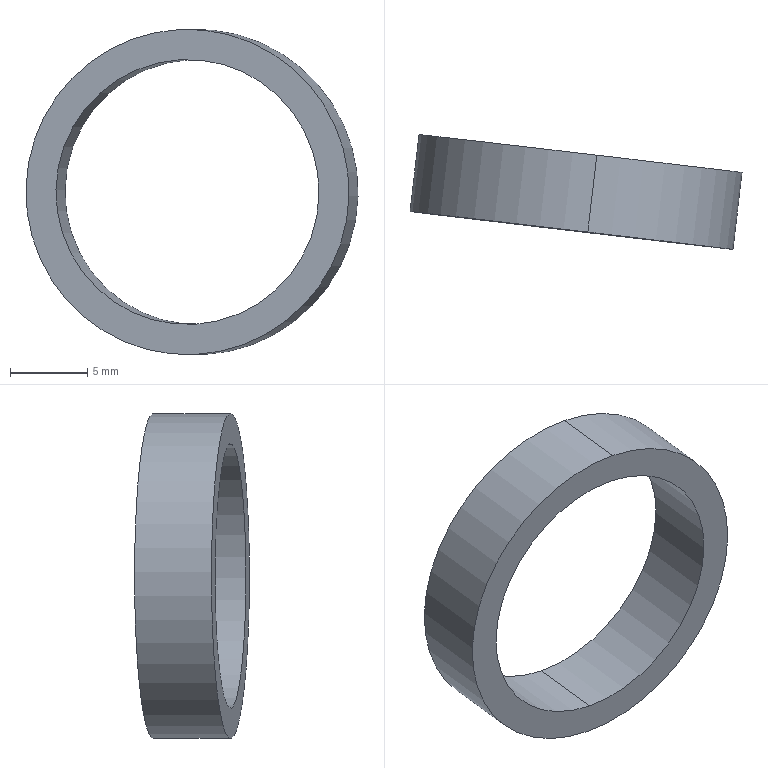Component | SolidWorks | 8TC-A17001-91-00UpperAndLowerPressAssembly-1_8TC-A17001-91-01Spacer-1 | 1 solid | 6 faces | box 21.44 x 7.42 x 21 mm | volume 584 mm3 | cylinder 4 | plane 2 | commonest cylinder face diameters 17.1 x2 21 x2 | material A3
build123d program:
from build123d import *

# Parameters (mm, degrees)
SKETCH1_R           = 10.5
SKETCH1_R_2         = 8.55
BOSS_EXTRUDE1_DEPTH = 5


with BuildPart() as part:
    # Sketch1 → Boss-Extrude1 (new body)
    with BuildSketch(Plane(origin=(0, 0, 0), x_dir=(1, 0, 0), z_dir=(0, 1, 0))):
        with Locations(Location((0, 0, 0), (0, 0, 270))):
            Circle(SKETCH1_R)
        with Locations(Location((0, 0, 0), (0, 0, 270))):
            Circle(SKETCH1_R_2, mode=Mode.SUBTRACT)
    extrude(amount=BOSS_EXTRUDE1_DEPTH)


solid = part.part

# Placed as in the assembly
solid = solid.moved(Location((1.253, -81.585, -52), (-35.549, -78.578, 143.907)))
STEP:
#1=CARTESIAN_POINT('',(0.0156,-3.208,-2.382));
#2=VERTEX_POINT('',#1);
#3=CARTESIAN_POINT('',(0.08309,-3.216,-1.712));
#4=VERTEX_POINT('',#3);
#5=CARTESIAN_POINT('',(0.04935,-3.212,-2.047));
#6=DIRECTION('',(0.1167,0.9932,-0.));
#7=DIRECTION('',(0.1002,-0.01178,0.9949));
#8=AXIS2_PLACEMENT_3D('',#5,#6,#7);
#9=CIRCLE('',#8,0.3366);
#10=EDGE_CURVE('',#2,#4,#9,.T.);
#11=ORIENTED_EDGE('',*,*,#10,.T.);
#12=CARTESIAN_POINT('',(0.06013,-3.411,-1.712));
#13=VERTEX_POINT('',#12);
#14=CARTESIAN_POINT('',(0.08309,-3.216,-1.712));
#15=DIRECTION('',(-0.1167,-0.9932,0.));
#16=VECTOR('',#15,39.37);
#17=LINE('',#14,#16);
#18=EDGE_CURVE('',#4,#13,#17,.T.);
#19=ORIENTED_EDGE('',*,*,#18,.T.);
#20=CARTESIAN_POINT('',(-0.007362,-3.404,-2.382));
#21=VERTEX_POINT('',#20);
#22=CARTESIAN_POINT('',(0.02638,-3.408,-2.047));
#23=DIRECTION('',(0.1167,0.9932,-0.));
#24=DIRECTION('',(0.1002,-0.01178,0.9949));
#25=AXIS2_PLACEMENT_3D('',#22,#23,#24);
#26=CIRCLE('',#25,0.3366);
#27=EDGE_CURVE('',#21,#13,#26,.T.);
#28=ORIENTED_EDGE('',*,*,#27,.F.);
#29=CARTESIAN_POINT('',(0.0156,-3.208,-2.382));
#30=DIRECTION('',(-0.1167,-0.9932,0.));
#31=VECTOR('',#30,39.37);
#32=LINE('',#29,#31);
#33=EDGE_CURVE('',#2,#21,#32,.T.);
#34=ORIENTED_EDGE('',*,*,#33,.F.);
#35=EDGE_LOOP('',(#11,#19,#28,#34));
#36=FACE_OUTER_BOUND('',#35,.T.);
#37=CARTESIAN_POINT('',(0.04935,-3.212,-2.047));
#38=DIRECTION('',(-0.1167,-0.9932,0.));
#39=DIRECTION('',(-0.1002,0.01178,-0.9949));
#40=AXIS2_PLACEMENT_3D('',#37,#38,#39);
#41=CYLINDRICAL_SURFACE('',#40,0.3366);
#42=ADVANCED_FACE('',(#36),#41,.F.);
#43=CARTESIAN_POINT('',(0.09079,-3.217,-1.636));
#44=VERTEX_POINT('',#43);
#45=CARTESIAN_POINT('',(0.007907,-3.207,-2.459));
#46=VERTEX_POINT('',#45);
#47=CARTESIAN_POINT('',(0.04935,-3.212,-2.047));
#48=DIRECTION('',(0.1167,0.9932,-0.));
#49=DIRECTION('',(0.1002,-0.01178,0.9949));
#50=AXIS2_PLACEMENT_3D('',#47,#48,#49);
#51=CIRCLE('',#50,0.4134);
#52=EDGE_CURVE('',#44,#46,#51,.T.);
#53=ORIENTED_EDGE('',*,*,#52,.F.);
#54=CARTESIAN_POINT('',(0.06782,-3.412,-1.636));
#55=VERTEX_POINT('',#54);
#56=CARTESIAN_POINT('',(0.09079,-3.217,-1.636));
#57=DIRECTION('',(-0.1167,-0.9932,0.));
#58=VECTOR('',#57,39.37);
#59=LINE('',#56,#58);
#60=EDGE_CURVE('',#44,#55,#59,.T.);
#61=ORIENTED_EDGE('',*,*,#60,.T.);
#62=CARTESIAN_POINT('',(-0.01506,-3.403,-2.459));
#63=VERTEX_POINT('',#62);
#64=CARTESIAN_POINT('',(0.02638,-3.408,-2.047));
#65=DIRECTION('',(0.1167,0.9932,-0.));
#66=DIRECTION('',(0.1002,-0.01178,0.9949));
#67=AXIS2_PLACEMENT_3D('',#64,#65,#66);
#68=CIRCLE('',#67,0.4134);
#69=EDGE_CURVE('',#55,#63,#68,.T.);
#70=ORIENTED_EDGE('',*,*,#69,.T.);
#71=CARTESIAN_POINT('',(0.007907,-3.207,-2.459));
#72=DIRECTION('',(-0.1167,-0.9932,0.));
#73=VECTOR('',#72,39.37);
#74=LINE('',#71,#73);
#75=EDGE_CURVE('',#46,#63,#74,.T.);
#76=ORIENTED_EDGE('',*,*,#75,.F.);
#77=EDGE_LOOP('',(#53,#61,#70,#76));
#78=FACE_OUTER_BOUND('',#77,.T.);
#79=CARTESIAN_POINT('',(0.04935,-3.212,-2.047));
#80=DIRECTION('',(-0.1167,-0.9932,0.));
#81=DIRECTION('',(-0.1002,0.01178,-0.9949));
#82=AXIS2_PLACEMENT_3D('',#79,#80,#81);
#83=CYLINDRICAL_SURFACE('',#82,0.4134);
#84=ADVANCED_FACE('',(#78),#83,.T.);
#85=CARTESIAN_POINT('',(0.04935,-3.212,-2.047));
#86=DIRECTION('',(0.1167,0.9932,-0.));
#87=DIRECTION('',(0.1002,-0.01178,0.9949));
#88=AXIS2_PLACEMENT_3D('',#85,#86,#87);
#89=CIRCLE('',#88,0.4134);
#90=EDGE_CURVE('',#46,#44,#89,.T.);
#91=ORIENTED_EDGE('',*,*,#90,.T.);
#92=ORIENTED_EDGE('',*,*,#52,.T.);
#93=EDGE_LOOP('',(#91,#92));
#94=FACE_OUTER_BOUND('',#93,.T.);
#95=ORIENTED_EDGE('',*,*,#10,.F.);
#96=CARTESIAN_POINT('',(0.04935,-3.212,-2.047));
#97=DIRECTION('',(0.1167,0.9932,-0.));
#98=DIRECTION('',(0.1002,-0.01178,0.9949));
#99=AXIS2_PLACEMENT_3D('',#96,#97,#98);
#100=CIRCLE('',#99,0.3366);
#101=EDGE_CURVE('',#4,#2,#100,.T.);
#102=ORIENTED_EDGE('',*,*,#101,.F.);
#103=EDGE_LOOP('',(#95,#102));
#104=FACE_BOUND('',#103,.T.);
#105=CARTESIAN_POINT('',(0.04935,-3.212,-2.047));
#106=DIRECTION('',(0.1167,0.9932,-0.));
#107=DIRECTION('',(0.1002,-0.01178,0.9949));
#108=AXIS2_PLACEMENT_3D('',#105,#106,#107);
#109=PLANE('',#108);
#110=ADVANCED_FACE('',(#94,#104),#109,.T.);
#111=CARTESIAN_POINT('',(0.02638,-3.408,-2.047));
#112=DIRECTION('',(0.1167,0.9932,-0.));
#113=DIRECTION('',(0.1002,-0.01178,0.9949));
#114=AXIS2_PLACEMENT_3D('',#111,#112,#113);
#115=CIRCLE('',#114,0.4134);
#116=EDGE_CURVE('',#63,#55,#115,.T.);
#117=ORIENTED_EDGE('',*,*,#116,.F.);
#118=ORIENTED_EDGE('',*,*,#69,.F.);
#119=EDGE_LOOP('',(#117,#118));
#120=FACE_OUTER_BOUND('',#119,.T.);
#121=ORIENTED_EDGE('',*,*,#27,.T.);
#122=CARTESIAN_POINT('',(0.02638,-3.408,-2.047));
#123=DIRECTION('',(0.1167,0.9932,-0.));
#124=DIRECTION('',(0.1002,-0.01178,0.9949));
#125=AXIS2_PLACEMENT_3D('',#122,#123,#124);
#126=CIRCLE('',#125,0.3366);
#127=EDGE_CURVE('',#13,#21,#126,.T.);
#128=ORIENTED_EDGE('',*,*,#127,.T.);
#129=EDGE_LOOP('',(#121,#128));
#130=FACE_BOUND('',#129,.T.);
#131=CARTESIAN_POINT('',(0.02638,-3.408,-2.047));
#132=DIRECTION('',(0.1167,0.9932,-0.));
#133=DIRECTION('',(0.1002,-0.01178,0.9949));
#134=AXIS2_PLACEMENT_3D('',#131,#132,#133);
#135=PLANE('',#134);
#136=ADVANCED_FACE('',(#120,#130),#135,.F.);
#137=ORIENTED_EDGE('',*,*,#60,.F.);
#138=ORIENTED_EDGE('',*,*,#90,.F.);
#139=ORIENTED_EDGE('',*,*,#75,.T.);
#140=ORIENTED_EDGE('',*,*,#116,.T.);
#141=EDGE_LOOP('',(#137,#138,#139,#140));
#142=FACE_OUTER_BOUND('',#141,.T.);
#143=CARTESIAN_POINT('',(0.04935,-3.212,-2.047));
#144=DIRECTION('',(-0.1167,-0.9932,0.));
#145=DIRECTION('',(-0.1002,0.01178,-0.9949));
#146=AXIS2_PLACEMENT_3D('',#143,#144,#145);
#147=CYLINDRICAL_SURFACE('',#146,0.4134);
#148=ADVANCED_FACE('',(#142),#147,.T.);
#149=ORIENTED_EDGE('',*,*,#18,.F.);
#150=ORIENTED_EDGE('',*,*,#101,.T.);
#151=ORIENTED_EDGE('',*,*,#33,.T.);
#152=ORIENTED_EDGE('',*,*,#127,.F.);
#153=EDGE_LOOP('',(#149,#150,#151,#152));
#154=FACE_OUTER_BOUND('',#153,.T.);
#155=CARTESIAN_POINT('',(0.04935,-3.212,-2.047));
#156=DIRECTION('',(-0.1167,-0.9932,0.));
#157=DIRECTION('',(-0.1002,0.01178,-0.9949));
#158=AXIS2_PLACEMENT_3D('',#155,#156,#157);
#159=CYLINDRICAL_SURFACE('',#158,0.3366);
#160=ADVANCED_FACE('',(#154),#159,.F.);
#161=CLOSED_SHELL('',(#42,#84,#110,#136,#148,#160));
#162=MANIFOLD_SOLID_BREP('',#161);
#163=CARTESIAN_POINT('',(0.,0.,0.));
#164=DIRECTION('',(0.,0.,1.));
#165=DIRECTION('',(1.,0.,0.));
#166=AXIS2_PLACEMENT_3D('',#163,#164,#165);
#167=(LENGTH_UNIT()NAMED_UNIT(*)SI_UNIT($,.METRE.));
#168=LENGTH_MEASURE_WITH_UNIT(LENGTH_MEASURE(0.0254),#167);
#169=DIMENSIONAL_EXPONENTS(1.,0.,0.,0.,0.,0.,0.);
#170=(CONVERSION_BASED_UNIT('',#168)LENGTH_UNIT()NAMED_UNIT(#169));
#171=UNCERTAINTY_MEASURE_WITH_UNIT(LENGTH_MEASURE(0.00001),#170,'','');
#172=(NAMED_UNIT(*)PLANE_ANGLE_UNIT()SI_UNIT($,.RADIAN.));
#173=(NAMED_UNIT(*)SI_UNIT($,.STERADIAN.)SOLID_ANGLE_UNIT());
#174=(GEOMETRIC_REPRESENTATION_CONTEXT(3)GLOBAL_UNCERTAINTY_ASSIGNED_CONTEXT((#171))GLOBAL_UNIT_ASSIGNED_CONTEXT((#170,#172,#173))REPRESENTATION_CONTEXT('',''));
#175=ADVANCED_BREP_SHAPE_REPRESENTATION('',(#162,#166),#174);
#176=COLOUR_RGB('',0.7922,0.8196,0.9333);
#177=FILL_AREA_STYLE_COLOUR('',#176);
#178=FILL_AREA_STYLE('',(#177));
#179=SURFACE_STYLE_FILL_AREA(#178);
#180=SURFACE_SIDE_STYLE('',(#179));
#181=SURFACE_STYLE_USAGE(.BOTH.,#180);
#182=PRESENTATION_STYLE_ASSIGNMENT((#181));
#183=STYLED_ITEM('',(#182),#162);
#184=(LENGTH_UNIT()NAMED_UNIT(*)SI_UNIT($,.METRE.));
#185=LENGTH_MEASURE_WITH_UNIT(LENGTH_MEASURE(0.0254),#184);
#186=DIMENSIONAL_EXPONENTS(1.,0.,0.,0.,0.,0.,0.);
#187=(CONVERSION_BASED_UNIT('',#185)LENGTH_UNIT()NAMED_UNIT(#186));
#188=UNCERTAINTY_MEASURE_WITH_UNIT(LENGTH_MEASURE(0.00001),#187,'','');
#189=(NAMED_UNIT(*)PLANE_ANGLE_UNIT()SI_UNIT($,.RADIAN.));
#190=(NAMED_UNIT(*)SI_UNIT($,.STERADIAN.)SOLID_ANGLE_UNIT());
#191=(GEOMETRIC_REPRESENTATION_CONTEXT(3)GLOBAL_UNCERTAINTY_ASSIGNED_CONTEXT((#188))GLOBAL_UNIT_ASSIGNED_CONTEXT((#187,#189,#190))REPRESENTATION_CONTEXT('',''));
#192=MECHANICAL_DESIGN_GEOMETRIC_PRESENTATION_REPRESENTATION('',(#183),#191);
#193=PRESENTATION_LAYER_ASSIGNMENT('','',(#183));